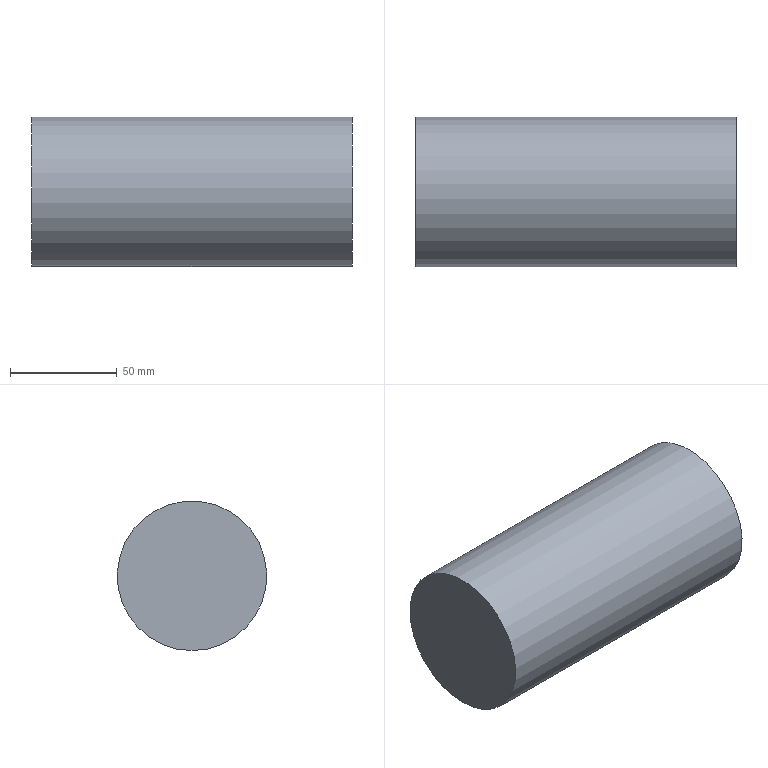Component | NX | SHAFT_PIN_70_150 | 1 solid | 3 faces | box 150 x 70 x 70 mm | volume 577268 mm3 | plane 2 | cylinder 1 | commonest cylinder face diameters 70 x1
STEP:
#1=CARTESIAN_POINT('',(0.,0.,0.));
#2=DIRECTION('',(0.,0.,1.));
#3=DIRECTION('',(1.,0.,0.));
#4=AXIS2_PLACEMENT_3D('',#1,#2,#3);
#5=CARTESIAN_POINT('',(-242.564,-997.61,-592.009));
#6=VERTEX_POINT('',#5);
#7=CARTESIAN_POINT('',(-242.564,-997.61,-557.009));
#8=DIRECTION('',(-1.,0.,0.));
#9=DIRECTION('',(0.,0.,-1.));
#10=AXIS2_PLACEMENT_3D('',#7,#8,#9);
#11=CIRCLE('',#10,35.);
#12=CARTESIAN_POINT('',(-242.564,-997.61,-557.009));
#13=DIRECTION('',(1.,0.,0.));
#14=DIRECTION('',(0.,0.,-1.));
#15=AXIS2_PLACEMENT_3D('',#12,#13,#14);
#16=PLANE('',#15);
#17=CARTESIAN_POINT('',(35.,0.));
#18=CARTESIAN_POINT('',(35.,-60.622));
#19=CARTESIAN_POINT('',(-17.5,-30.311));
#20=CARTESIAN_POINT('',(-70.,-0.));
#21=CARTESIAN_POINT('',(-17.5,30.311));
#22=CARTESIAN_POINT('',(35.,60.622));
#23=CARTESIAN_POINT('',(35.,0.));
#24=(BOUNDED_CURVE()B_SPLINE_CURVE(2,(#17,#18,#19,#20,#21,#22,#23),.UNSPECIFIED.,.T.,.F.)B_SPLINE_CURVE_WITH_KNOTS((1,2,2,2,2,1),(-2.094,0.,2.094,4.189,6.283,8.378),.UNSPECIFIED.)CURVE()GEOMETRIC_REPRESENTATION_ITEM()RATIONAL_B_SPLINE_CURVE((1.,0.5,1.,0.5,1.,0.5,1.))REPRESENTATION_ITEM(''));
#25=(GEOMETRIC_REPRESENTATION_CONTEXT(2)PARAMETRIC_REPRESENTATION_CONTEXT()REPRESENTATION_CONTEXT('',''));
#26=DEFINITIONAL_REPRESENTATION('',(#24),#25);
#27=PCURVE('',#16,#26);
#28=CARTESIAN_POINT('',(-392.564,-997.61,-557.009));
#29=DIRECTION('',(1.,0.,0.));
#30=DIRECTION('',(0.,0.,-1.));
#31=AXIS2_PLACEMENT_3D('',#28,#29,#30);
#32=CYLINDRICAL_SURFACE('',#31,35.);
#33=CARTESIAN_POINT('',(6.283,150.));
#34=DIRECTION('',(-1.,0.));
#35=VECTOR('',#34,1.);
#36=LINE('',#33,#35);
#37=(GEOMETRIC_REPRESENTATION_CONTEXT(2)PARAMETRIC_REPRESENTATION_CONTEXT()REPRESENTATION_CONTEXT('',''));
#38=DEFINITIONAL_REPRESENTATION('',(#36),#37);
#39=PCURVE('',#32,#38);
#40=SURFACE_CURVE('',#11,(#27,#39),.PCURVE_S1.);
#41=EDGE_CURVE('',#6,#6,#40,.T.);
#42=ORIENTED_EDGE('',*,*,#41,.F.);
#43=EDGE_LOOP('',(#42));
#44=FACE_BOUND('',#43,.T.);
#45=ADVANCED_FACE('',(#44),#16,.T.);
#46=CARTESIAN_POINT('',(-392.564,-997.61,-592.009));
#47=VERTEX_POINT('',#46);
#48=CARTESIAN_POINT('',(-392.564,-997.61,-557.009));
#49=DIRECTION('',(1.,0.,0.));
#50=DIRECTION('',(0.,0.,-1.));
#51=AXIS2_PLACEMENT_3D('',#48,#49,#50);
#52=CIRCLE('',#51,35.);
#53=CARTESIAN_POINT('',(-392.564,-997.61,-557.009));
#54=DIRECTION('',(-1.,0.,0.));
#55=DIRECTION('',(0.,0.,1.));
#56=AXIS2_PLACEMENT_3D('',#53,#54,#55);
#57=PLANE('',#56);
#58=CARTESIAN_POINT('',(-35.,0.));
#59=CARTESIAN_POINT('',(-35.,60.622));
#60=CARTESIAN_POINT('',(17.5,30.311));
#61=CARTESIAN_POINT('',(70.,0.));
#62=CARTESIAN_POINT('',(17.5,-30.311));
#63=CARTESIAN_POINT('',(-35.,-60.622));
#64=CARTESIAN_POINT('',(-35.,0.));
#65=(BOUNDED_CURVE()B_SPLINE_CURVE(2,(#58,#59,#60,#61,#62,#63,#64),.UNSPECIFIED.,.T.,.F.)B_SPLINE_CURVE_WITH_KNOTS((1,2,2,2,2,1),(-2.094,0.,2.094,4.189,6.283,8.378),.UNSPECIFIED.)CURVE()GEOMETRIC_REPRESENTATION_ITEM()RATIONAL_B_SPLINE_CURVE((1.,0.5,1.,0.5,1.,0.5,1.))REPRESENTATION_ITEM(''));
#66=(GEOMETRIC_REPRESENTATION_CONTEXT(2)PARAMETRIC_REPRESENTATION_CONTEXT()REPRESENTATION_CONTEXT('',''));
#67=DEFINITIONAL_REPRESENTATION('',(#65),#66);
#68=PCURVE('',#57,#67);
#69=CARTESIAN_POINT('',(0.,0.));
#70=DIRECTION('',(1.,0.));
#71=VECTOR('',#70,1.);
#72=LINE('',#69,#71);
#73=(GEOMETRIC_REPRESENTATION_CONTEXT(2)PARAMETRIC_REPRESENTATION_CONTEXT()REPRESENTATION_CONTEXT('',''));
#74=DEFINITIONAL_REPRESENTATION('',(#72),#73);
#75=PCURVE('',#32,#74);
#76=SURFACE_CURVE('',#52,(#68,#75),.PCURVE_S1.);
#77=EDGE_CURVE('',#47,#47,#76,.T.);
#78=ORIENTED_EDGE('',*,*,#77,.F.);
#79=EDGE_LOOP('',(#78));
#80=FACE_BOUND('',#79,.T.);
#81=ADVANCED_FACE('',(#80),#57,.T.);
#82=ORIENTED_EDGE('',*,*,#41,.T.);
#83=CARTESIAN_POINT('',(-392.564,-997.61,-592.009));
#84=CARTESIAN_POINT('',(-242.564,-997.61,-592.009));
#85=B_SPLINE_CURVE_WITH_KNOTS('',1,(#83,#84),.UNSPECIFIED.,.F.,.F.,(2,2),(0.,150.),.PIECEWISE_BEZIER_KNOTS.);
#86=CARTESIAN_POINT('',(0.,0.));
#87=DIRECTION('',(0.,1.));
#88=VECTOR('',#87,1.);
#89=LINE('',#86,#88);
#90=(GEOMETRIC_REPRESENTATION_CONTEXT(2)PARAMETRIC_REPRESENTATION_CONTEXT()REPRESENTATION_CONTEXT('',''));
#91=DEFINITIONAL_REPRESENTATION('',(#89),#90);
#92=PCURVE('',#32,#91);
#93=CARTESIAN_POINT('',(6.283,0.));
#94=DIRECTION('',(0.,1.));
#95=VECTOR('',#94,1.);
#96=LINE('',#93,#95);
#97=(GEOMETRIC_REPRESENTATION_CONTEXT(2)PARAMETRIC_REPRESENTATION_CONTEXT()REPRESENTATION_CONTEXT('',''));
#98=DEFINITIONAL_REPRESENTATION('',(#96),#97);
#99=PCURVE('',#32,#98);
#100=SEAM_CURVE('',#85,(#92,#99),.PCURVE_S1.);
#101=EDGE_CURVE('',#47,#6,#100,.T.);
#102=ORIENTED_EDGE('',*,*,#101,.F.);
#103=ORIENTED_EDGE('',*,*,#77,.T.);
#104=ORIENTED_EDGE('',*,*,#101,.T.);
#105=EDGE_LOOP('',(#82,#102,#103,#104));
#106=FACE_BOUND('',#105,.T.);
#107=ADVANCED_FACE('',(#106),#32,.T.);
#108=CLOSED_SHELL('',(#45,#81,#107));
#109=MANIFOLD_SOLID_BREP('',#108);
#110=(LENGTH_UNIT()NAMED_UNIT(*)SI_UNIT(.MILLI.,.METRE.));
#111=UNCERTAINTY_MEASURE_WITH_UNIT(LENGTH_MEASURE(0.00001),#110,'','');
#112=(NAMED_UNIT(*)PLANE_ANGLE_UNIT()SI_UNIT($,.RADIAN.));
#113=(NAMED_UNIT(*)SI_UNIT($,.STERADIAN.)SOLID_ANGLE_UNIT());
#114=(GEOMETRIC_REPRESENTATION_CONTEXT(3)GLOBAL_UNCERTAINTY_ASSIGNED_CONTEXT((#111))GLOBAL_UNIT_ASSIGNED_CONTEXT((#110,#112,#113))REPRESENTATION_CONTEXT('',''));
#115=ADVANCED_BREP_SHAPE_REPRESENTATION('',(#4,#109),#114);